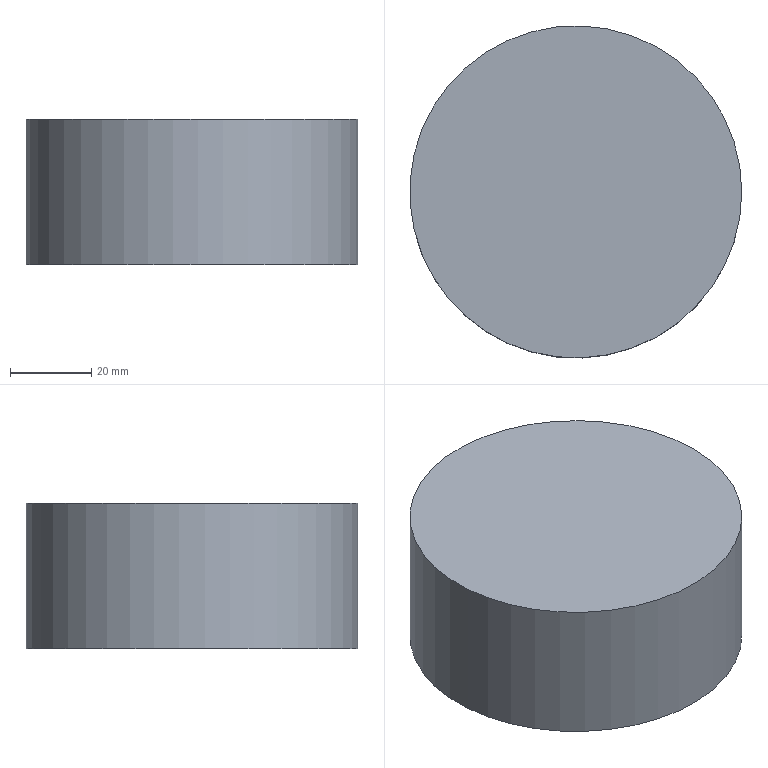Component | NX | SCREW_PLUG | 1 solid | 7 faces | box 81.95 x 81.95 x 36 mm | volume 189778 mm3 | cylinder 3 | plane 2 | cone 2 | commonest cylinder face diameters 4 x2 81.945 x1
STEP:
#1=CARTESIAN_POINT('',(0.,0.,0.));
#2=DIRECTION('',(0.,0.,1.));
#3=DIRECTION('',(1.,0.,0.));
#4=AXIS2_PLACEMENT_3D('',#1,#2,#3);
#5=CARTESIAN_POINT('',(122.222,-116.649,-169.615));
#6=VERTEX_POINT('',#5);
#7=CARTESIAN_POINT('',(81.249,-116.649,-169.615));
#8=DIRECTION('',(0.,0.,-1.));
#9=DIRECTION('',(1.,0.,0.));
#10=AXIS2_PLACEMENT_3D('',#7,#8,#9);
#11=CIRCLE('',#10,40.973);
#12=CARTESIAN_POINT('',(81.249,-116.649,-169.615));
#13=DIRECTION('',(0.,0.,1.));
#14=DIRECTION('',(1.,0.,0.));
#15=AXIS2_PLACEMENT_3D('',#12,#13,#14);
#16=PLANE('',#15);
#17=CARTESIAN_POINT('',(40.973,0.));
#18=CARTESIAN_POINT('',(40.973,-70.967));
#19=CARTESIAN_POINT('',(-20.486,-35.483));
#20=CARTESIAN_POINT('',(-81.945,-0.));
#21=CARTESIAN_POINT('',(-20.486,35.483));
#22=CARTESIAN_POINT('',(40.973,70.967));
#23=CARTESIAN_POINT('',(40.973,0.));
#24=(BOUNDED_CURVE()B_SPLINE_CURVE(2,(#17,#18,#19,#20,#21,#22,#23),.UNSPECIFIED.,.T.,.F.)B_SPLINE_CURVE_WITH_KNOTS((1,2,2,2,2,1),(-2.094,0.,2.094,4.189,6.283,8.378),.UNSPECIFIED.)CURVE()GEOMETRIC_REPRESENTATION_ITEM()RATIONAL_B_SPLINE_CURVE((1.,0.5,1.,0.5,1.,0.5,1.))REPRESENTATION_ITEM(''));
#25=(GEOMETRIC_REPRESENTATION_CONTEXT(2)PARAMETRIC_REPRESENTATION_CONTEXT()REPRESENTATION_CONTEXT('',''));
#26=DEFINITIONAL_REPRESENTATION('',(#24),#25);
#27=PCURVE('',#16,#26);
#28=CARTESIAN_POINT('',(81.249,-116.649,-205.615));
#29=DIRECTION('',(0.,0.,1.));
#30=DIRECTION('',(1.,0.,0.));
#31=AXIS2_PLACEMENT_3D('',#28,#29,#30);
#32=CYLINDRICAL_SURFACE('',#31,40.973);
#33=CARTESIAN_POINT('',(6.283,36.));
#34=DIRECTION('',(-1.,0.));
#35=VECTOR('',#34,1.);
#36=LINE('',#33,#35);
#37=(GEOMETRIC_REPRESENTATION_CONTEXT(2)PARAMETRIC_REPRESENTATION_CONTEXT()REPRESENTATION_CONTEXT('',''));
#38=DEFINITIONAL_REPRESENTATION('',(#36),#37);
#39=PCURVE('',#32,#38);
#40=SURFACE_CURVE('',#11,(#27,#39),.PCURVE_S1.);
#41=EDGE_CURVE('',#6,#6,#40,.T.);
#42=ORIENTED_EDGE('',*,*,#41,.F.);
#43=EDGE_LOOP('',(#42));
#44=FACE_BOUND('',#43,.T.);
#45=ADVANCED_FACE('',(#44),#16,.T.);
#46=CARTESIAN_POINT('',(62.999,-116.649,-205.615));
#47=VERTEX_POINT('',#46);
#48=CARTESIAN_POINT('',(60.999,-116.649,-205.615));
#49=DIRECTION('',(0.,0.,1.));
#50=DIRECTION('',(1.,0.,0.));
#51=AXIS2_PLACEMENT_3D('',#48,#49,#50);
#52=CIRCLE('',#51,2.);
#53=CARTESIAN_POINT('',(81.249,-116.649,-205.615));
#54=DIRECTION('',(0.,0.,-1.));
#55=DIRECTION('',(-1.,0.,0.));
#56=AXIS2_PLACEMENT_3D('',#53,#54,#55);
#57=PLANE('',#56);
#58=CARTESIAN_POINT('',(18.25,0.));
#59=CARTESIAN_POINT('',(18.25,3.464));
#60=CARTESIAN_POINT('',(21.25,1.732));
#61=CARTESIAN_POINT('',(24.25,0.));
#62=CARTESIAN_POINT('',(21.25,-1.732));
#63=CARTESIAN_POINT('',(18.25,-3.464));
#64=CARTESIAN_POINT('',(18.25,0.));
#65=(BOUNDED_CURVE()B_SPLINE_CURVE(2,(#58,#59,#60,#61,#62,#63,#64),.UNSPECIFIED.,.T.,.F.)B_SPLINE_CURVE_WITH_KNOTS((1,2,2,2,2,1),(-2.094,0.,2.094,4.189,6.283,8.378),.UNSPECIFIED.)CURVE()GEOMETRIC_REPRESENTATION_ITEM()RATIONAL_B_SPLINE_CURVE((1.,0.5,1.,0.5,1.,0.5,1.))REPRESENTATION_ITEM(''));
#66=(GEOMETRIC_REPRESENTATION_CONTEXT(2)PARAMETRIC_REPRESENTATION_CONTEXT()REPRESENTATION_CONTEXT('',''));
#67=DEFINITIONAL_REPRESENTATION('',(#65),#66);
#68=PCURVE('',#57,#67);
#69=CARTESIAN_POINT('',(60.999,-116.649,-205.615));
#70=DIRECTION('',(0.,0.,1.));
#71=DIRECTION('',(1.,0.,0.));
#72=AXIS2_PLACEMENT_3D('',#69,#70,#71);
#73=CYLINDRICAL_SURFACE('',#72,2.);
#74=CARTESIAN_POINT('',(0.,0.));
#75=DIRECTION('',(1.,0.));
#76=VECTOR('',#75,1.);
#77=LINE('',#74,#76);
#78=(GEOMETRIC_REPRESENTATION_CONTEXT(2)PARAMETRIC_REPRESENTATION_CONTEXT()REPRESENTATION_CONTEXT('',''));
#79=DEFINITIONAL_REPRESENTATION('',(#77),#78);
#80=PCURVE('',#73,#79);
#81=SURFACE_CURVE('',#52,(#68,#80),.PCURVE_S1.);
#82=EDGE_CURVE('',#47,#47,#81,.T.);
#83=ORIENTED_EDGE('',*,*,#82,.T.);
#84=EDGE_LOOP('',(#83));
#85=FACE_BOUND('',#84,.T.);
#86=CARTESIAN_POINT('',(103.499,-116.649,-205.615));
#87=VERTEX_POINT('',#86);
#88=CARTESIAN_POINT('',(101.499,-116.649,-205.615));
#89=DIRECTION('',(0.,0.,1.));
#90=DIRECTION('',(1.,0.,0.));
#91=AXIS2_PLACEMENT_3D('',#88,#89,#90);
#92=CIRCLE('',#91,2.);
#93=CARTESIAN_POINT('',(-22.25,0.));
#94=CARTESIAN_POINT('',(-22.25,3.464));
#95=CARTESIAN_POINT('',(-19.25,1.732));
#96=CARTESIAN_POINT('',(-16.25,0.));
#97=CARTESIAN_POINT('',(-19.25,-1.732));
#98=CARTESIAN_POINT('',(-22.25,-3.464));
#99=CARTESIAN_POINT('',(-22.25,0.));
#100=(BOUNDED_CURVE()B_SPLINE_CURVE(2,(#93,#94,#95,#96,#97,#98,#99),.UNSPECIFIED.,.T.,.F.)B_SPLINE_CURVE_WITH_KNOTS((1,2,2,2,2,1),(-2.094,0.,2.094,4.189,6.283,8.378),.UNSPECIFIED.)CURVE()GEOMETRIC_REPRESENTATION_ITEM()RATIONAL_B_SPLINE_CURVE((1.,0.5,1.,0.5,1.,0.5,1.))REPRESENTATION_ITEM(''));
#101=(GEOMETRIC_REPRESENTATION_CONTEXT(2)PARAMETRIC_REPRESENTATION_CONTEXT()REPRESENTATION_CONTEXT('',''));
#102=DEFINITIONAL_REPRESENTATION('',(#100),#101);
#103=PCURVE('',#57,#102);
#104=CARTESIAN_POINT('',(101.499,-116.649,-205.615));
#105=DIRECTION('',(0.,0.,1.));
#106=DIRECTION('',(1.,0.,0.));
#107=AXIS2_PLACEMENT_3D('',#104,#105,#106);
#108=CYLINDRICAL_SURFACE('',#107,2.);
#109=CARTESIAN_POINT('',(0.,0.));
#110=DIRECTION('',(1.,0.));
#111=VECTOR('',#110,1.);
#112=LINE('',#109,#111);
#113=(GEOMETRIC_REPRESENTATION_CONTEXT(2)PARAMETRIC_REPRESENTATION_CONTEXT()REPRESENTATION_CONTEXT('',''));
#114=DEFINITIONAL_REPRESENTATION('',(#112),#113);
#115=PCURVE('',#108,#114);
#116=SURFACE_CURVE('',#92,(#103,#115),.PCURVE_S1.);
#117=EDGE_CURVE('',#87,#87,#116,.T.);
#118=ORIENTED_EDGE('',*,*,#117,.T.);
#119=EDGE_LOOP('',(#118));
#120=FACE_BOUND('',#119,.T.);
#121=CARTESIAN_POINT('',(122.222,-116.649,-205.615));
#122=VERTEX_POINT('',#121);
#123=CARTESIAN_POINT('',(81.249,-116.649,-205.615));
#124=DIRECTION('',(0.,0.,1.));
#125=DIRECTION('',(1.,0.,0.));
#126=AXIS2_PLACEMENT_3D('',#123,#124,#125);
#127=CIRCLE('',#126,40.973);
#128=CARTESIAN_POINT('',(-40.973,0.));
#129=CARTESIAN_POINT('',(-40.973,70.967));
#130=CARTESIAN_POINT('',(20.486,35.483));
#131=CARTESIAN_POINT('',(81.945,0.));
#132=CARTESIAN_POINT('',(20.486,-35.483));
#133=CARTESIAN_POINT('',(-40.973,-70.967));
#134=CARTESIAN_POINT('',(-40.973,0.));
#135=(BOUNDED_CURVE()B_SPLINE_CURVE(2,(#128,#129,#130,#131,#132,#133,#134),.UNSPECIFIED.,.T.,.F.)B_SPLINE_CURVE_WITH_KNOTS((1,2,2,2,2,1),(-2.094,0.,2.094,4.189,6.283,8.378),.UNSPECIFIED.)CURVE()GEOMETRIC_REPRESENTATION_ITEM()RATIONAL_B_SPLINE_CURVE((1.,0.5,1.,0.5,1.,0.5,1.))REPRESENTATION_ITEM(''));
#136=(GEOMETRIC_REPRESENTATION_CONTEXT(2)PARAMETRIC_REPRESENTATION_CONTEXT()REPRESENTATION_CONTEXT('',''));
#137=DEFINITIONAL_REPRESENTATION('',(#135),#136);
#138=PCURVE('',#57,#137);
#139=CARTESIAN_POINT('',(0.,0.));
#140=DIRECTION('',(1.,0.));
#141=VECTOR('',#140,1.);
#142=LINE('',#139,#141);
#143=(GEOMETRIC_REPRESENTATION_CONTEXT(2)PARAMETRIC_REPRESENTATION_CONTEXT()REPRESENTATION_CONTEXT('',''));
#144=DEFINITIONAL_REPRESENTATION('',(#142),#143);
#145=PCURVE('',#32,#144);
#146=SURFACE_CURVE('',#127,(#138,#145),.PCURVE_S1.);
#147=EDGE_CURVE('',#122,#122,#146,.T.);
#148=ORIENTED_EDGE('',*,*,#147,.F.);
#149=EDGE_LOOP('',(#148));
#150=FACE_BOUND('',#149,.T.);
#151=ADVANCED_FACE('',(#85,#120,#150),#57,.T.);
#152=ORIENTED_EDGE('',*,*,#41,.T.);
#153=CARTESIAN_POINT('',(122.222,-116.649,-205.615));
#154=CARTESIAN_POINT('',(122.222,-116.649,-169.615));
#155=B_SPLINE_CURVE_WITH_KNOTS('',1,(#153,#154),.UNSPECIFIED.,.F.,.F.,(2,2),(0.,36.),.PIECEWISE_BEZIER_KNOTS.);
#156=CARTESIAN_POINT('',(0.,0.));
#157=DIRECTION('',(0.,1.));
#158=VECTOR('',#157,1.);
#159=LINE('',#156,#158);
#160=(GEOMETRIC_REPRESENTATION_CONTEXT(2)PARAMETRIC_REPRESENTATION_CONTEXT()REPRESENTATION_CONTEXT('',''));
#161=DEFINITIONAL_REPRESENTATION('',(#159),#160);
#162=PCURVE('',#32,#161);
#163=CARTESIAN_POINT('',(6.283,0.));
#164=DIRECTION('',(0.,1.));
#165=VECTOR('',#164,1.);
#166=LINE('',#163,#165);
#167=(GEOMETRIC_REPRESENTATION_CONTEXT(2)PARAMETRIC_REPRESENTATION_CONTEXT()REPRESENTATION_CONTEXT('',''));
#168=DEFINITIONAL_REPRESENTATION('',(#166),#167);
#169=PCURVE('',#32,#168);
#170=SEAM_CURVE('',#155,(#162,#169),.PCURVE_S1.);
#171=EDGE_CURVE('',#122,#6,#170,.T.);
#172=ORIENTED_EDGE('',*,*,#171,.F.);
#173=ORIENTED_EDGE('',*,*,#147,.T.);
#174=ORIENTED_EDGE('',*,*,#171,.T.);
#175=EDGE_LOOP('',(#152,#172,#173,#174));
#176=FACE_BOUND('',#175,.T.);
#177=ADVANCED_FACE('',(#176),#32,.T.);
#178=CARTESIAN_POINT('',(99.499,-116.649,-202.615));
#179=VERTEX_POINT('',#178);
#180=CARTESIAN_POINT('',(103.499,-116.649,-202.615));
#181=VERTEX_POINT('',#180);
#182=CARTESIAN_POINT('',(101.499,-116.649,-202.615));
#183=DIRECTION('',(0.,0.,-1.));
#184=DIRECTION('',(1.,0.,0.));
#185=AXIS2_PLACEMENT_3D('',#182,#183,#184);
#186=CIRCLE('',#185,2.);
#187=CARTESIAN_POINT('',(101.499,-116.649,-202.615));
#188=DIRECTION('',(0.,0.,-1.));
#189=DIRECTION('',(-1.,0.,0.));
#190=AXIS2_PLACEMENT_3D('',#187,#188,#189);
#191=CONICAL_SURFACE('',#190,2.,1.03);
#192=CARTESIAN_POINT('',(-3.142,0.));
#193=DIRECTION('',(1.,0.));
#194=VECTOR('',#193,1.);
#195=LINE('',#192,#194);
#196=(GEOMETRIC_REPRESENTATION_CONTEXT(2)PARAMETRIC_REPRESENTATION_CONTEXT()REPRESENTATION_CONTEXT('',''));
#197=DEFINITIONAL_REPRESENTATION('',(#195),#196);
#198=PCURVE('',#191,#197);
#199=CARTESIAN_POINT('',(6.283,3.));
#200=DIRECTION('',(-1.,0.));
#201=VECTOR('',#200,1.);
#202=LINE('',#199,#201);
#203=(GEOMETRIC_REPRESENTATION_CONTEXT(2)PARAMETRIC_REPRESENTATION_CONTEXT()REPRESENTATION_CONTEXT('',''));
#204=DEFINITIONAL_REPRESENTATION('',(#202),#203);
#205=PCURVE('',#108,#204);
#206=SURFACE_CURVE('',#186,(#198,#205),.PCURVE_S1.);
#207=EDGE_CURVE('',#179,#181,#206,.T.);
#208=ORIENTED_EDGE('',*,*,#207,.F.);
#209=CARTESIAN_POINT('',(101.499,-116.649,-201.413));
#210=VERTEX_POINT('',#209);
#211=CARTESIAN_POINT('',(101.499,-116.649,-201.413));
#212=CARTESIAN_POINT('',(99.499,-116.649,-202.615));
#213=B_SPLINE_CURVE_WITH_KNOTS('',1,(#211,#212),.UNSPECIFIED.,.F.,.F.,(2,2),(-2.333,0.),.PIECEWISE_BEZIER_KNOTS.);
#214=CARTESIAN_POINT('',(0.,0.));
#215=DIRECTION('',(0.,1.));
#216=VECTOR('',#215,1.);
#217=LINE('',#214,#216);
#218=(GEOMETRIC_REPRESENTATION_CONTEXT(2)PARAMETRIC_REPRESENTATION_CONTEXT()REPRESENTATION_CONTEXT('',''));
#219=DEFINITIONAL_REPRESENTATION('',(#217),#218);
#220=PCURVE('',#191,#219);
#221=CARTESIAN_POINT('',(6.283,0.));
#222=DIRECTION('',(0.,1.));
#223=VECTOR('',#222,1.);
#224=LINE('',#221,#223);
#225=(GEOMETRIC_REPRESENTATION_CONTEXT(2)PARAMETRIC_REPRESENTATION_CONTEXT()REPRESENTATION_CONTEXT('',''));
#226=DEFINITIONAL_REPRESENTATION('',(#224),#225);
#227=PCURVE('',#191,#226);
#228=SEAM_CURVE('',#213,(#220,#227),.PCURVE_S1.);
#229=EDGE_CURVE('',#210,#179,#228,.T.);
#230=ORIENTED_EDGE('',*,*,#229,.F.);
#231=ORIENTED_EDGE('',*,*,#229,.T.);
#232=CARTESIAN_POINT('',(101.499,-116.649,-202.615));
#233=DIRECTION('',(0.,0.,-1.));
#234=DIRECTION('',(1.,0.,0.));
#235=AXIS2_PLACEMENT_3D('',#232,#233,#234);
#236=CIRCLE('',#235,2.);
#237=CARTESIAN_POINT('',(3.142,0.));
#238=DIRECTION('',(1.,0.));
#239=VECTOR('',#238,1.);
#240=LINE('',#237,#239);
#241=(GEOMETRIC_REPRESENTATION_CONTEXT(2)PARAMETRIC_REPRESENTATION_CONTEXT()REPRESENTATION_CONTEXT('',''));
#242=DEFINITIONAL_REPRESENTATION('',(#240),#241);
#243=PCURVE('',#191,#242);
#244=CARTESIAN_POINT('',(6.283,3.));
#245=DIRECTION('',(-1.,0.));
#246=VECTOR('',#245,1.);
#247=LINE('',#244,#246);
#248=(GEOMETRIC_REPRESENTATION_CONTEXT(2)PARAMETRIC_REPRESENTATION_CONTEXT()REPRESENTATION_CONTEXT('',''));
#249=DEFINITIONAL_REPRESENTATION('',(#247),#248);
#250=PCURVE('',#108,#249);
#251=SURFACE_CURVE('',#236,(#243,#250),.PCURVE_S1.);
#252=EDGE_CURVE('',#181,#179,#251,.T.);
#253=ORIENTED_EDGE('',*,*,#252,.F.);
#254=EDGE_LOOP('',(#208,#230,#231,#253));
#255=FACE_BOUND('',#254,.F.);
#256=ADVANCED_FACE('',(#255),#191,.F.);
#257=ORIENTED_EDGE('',*,*,#207,.T.);
#258=CARTESIAN_POINT('',(103.499,-116.649,-205.615));
#259=CARTESIAN_POINT('',(103.499,-116.649,-202.615));
#260=B_SPLINE_CURVE_WITH_KNOTS('',1,(#258,#259),.UNSPECIFIED.,.F.,.F.,(2,2),(0.,3.),.PIECEWISE_BEZIER_KNOTS.);
#261=CARTESIAN_POINT('',(0.,0.));
#262=DIRECTION('',(0.,1.));
#263=VECTOR('',#262,1.);
#264=LINE('',#261,#263);
#265=(GEOMETRIC_REPRESENTATION_CONTEXT(2)PARAMETRIC_REPRESENTATION_CONTEXT()REPRESENTATION_CONTEXT('',''));
#266=DEFINITIONAL_REPRESENTATION('',(#264),#265);
#267=PCURVE('',#108,#266);
#268=CARTESIAN_POINT('',(6.283,0.));
#269=DIRECTION('',(0.,1.));
#270=VECTOR('',#269,1.);
#271=LINE('',#268,#270);
#272=(GEOMETRIC_REPRESENTATION_CONTEXT(2)PARAMETRIC_REPRESENTATION_CONTEXT()REPRESENTATION_CONTEXT('',''));
#273=DEFINITIONAL_REPRESENTATION('',(#271),#272);
#274=PCURVE('',#108,#273);
#275=SEAM_CURVE('',#260,(#267,#274),.PCURVE_S1.);
#276=EDGE_CURVE('',#87,#181,#275,.T.);
#277=ORIENTED_EDGE('',*,*,#276,.F.);
#278=ORIENTED_EDGE('',*,*,#117,.T.);
#279=ORIENTED_EDGE('',*,*,#276,.T.);
#280=ORIENTED_EDGE('',*,*,#252,.T.);
#281=EDGE_LOOP('',(#257,#277,#278,#279,#280));
#282=FACE_BOUND('',#281,.F.);
#283=ADVANCED_FACE('',(#282),#108,.F.);
#284=CARTESIAN_POINT('',(58.999,-116.649,-202.615));
#285=VERTEX_POINT('',#284);
#286=CARTESIAN_POINT('',(62.999,-116.649,-202.615));
#287=VERTEX_POINT('',#286);
#288=CARTESIAN_POINT('',(60.999,-116.649,-202.615));
#289=DIRECTION('',(0.,0.,-1.));
#290=DIRECTION('',(1.,0.,0.));
#291=AXIS2_PLACEMENT_3D('',#288,#289,#290);
#292=CIRCLE('',#291,2.);
#293=CARTESIAN_POINT('',(60.999,-116.649,-202.615));
#294=DIRECTION('',(0.,0.,-1.));
#295=DIRECTION('',(-1.,0.,0.));
#296=AXIS2_PLACEMENT_3D('',#293,#294,#295);
#297=CONICAL_SURFACE('',#296,2.,1.03);
#298=CARTESIAN_POINT('',(-3.142,0.));
#299=DIRECTION('',(1.,0.));
#300=VECTOR('',#299,1.);
#301=LINE('',#298,#300);
#302=(GEOMETRIC_REPRESENTATION_CONTEXT(2)PARAMETRIC_REPRESENTATION_CONTEXT()REPRESENTATION_CONTEXT('',''));
#303=DEFINITIONAL_REPRESENTATION('',(#301),#302);
#304=PCURVE('',#297,#303);
#305=CARTESIAN_POINT('',(6.283,3.));
#306=DIRECTION('',(-1.,0.));
#307=VECTOR('',#306,1.);
#308=LINE('',#305,#307);
#309=(GEOMETRIC_REPRESENTATION_CONTEXT(2)PARAMETRIC_REPRESENTATION_CONTEXT()REPRESENTATION_CONTEXT('',''));
#310=DEFINITIONAL_REPRESENTATION('',(#308),#309);
#311=PCURVE('',#73,#310);
#312=SURFACE_CURVE('',#292,(#304,#311),.PCURVE_S1.);
#313=EDGE_CURVE('',#285,#287,#312,.T.);
#314=ORIENTED_EDGE('',*,*,#313,.F.);
#315=CARTESIAN_POINT('',(60.999,-116.649,-201.413));
#316=VERTEX_POINT('',#315);
#317=CARTESIAN_POINT('',(60.999,-116.649,-201.413));
#318=CARTESIAN_POINT('',(58.999,-116.649,-202.615));
#319=B_SPLINE_CURVE_WITH_KNOTS('',1,(#317,#318),.UNSPECIFIED.,.F.,.F.,(2,2),(-2.333,0.),.PIECEWISE_BEZIER_KNOTS.);
#320=CARTESIAN_POINT('',(0.,0.));
#321=DIRECTION('',(0.,1.));
#322=VECTOR('',#321,1.);
#323=LINE('',#320,#322);
#324=(GEOMETRIC_REPRESENTATION_CONTEXT(2)PARAMETRIC_REPRESENTATION_CONTEXT()REPRESENTATION_CONTEXT('',''));
#325=DEFINITIONAL_REPRESENTATION('',(#323),#324);
#326=PCURVE('',#297,#325);
#327=CARTESIAN_POINT('',(6.283,0.));
#328=DIRECTION('',(0.,1.));
#329=VECTOR('',#328,1.);
#330=LINE('',#327,#329);
#331=(GEOMETRIC_REPRESENTATION_CONTEXT(2)PARAMETRIC_REPRESENTATION_CONTEXT()REPRESENTATION_CONTEXT('',''));
#332=DEFINITIONAL_REPRESENTATION('',(#330),#331);
#333=PCURVE('',#297,#332);
#334=SEAM_CURVE('',#319,(#326,#333),.PCURVE_S1.);
#335=EDGE_CURVE('',#316,#285,#334,.T.);
#336=ORIENTED_EDGE('',*,*,#335,.F.);
#337=ORIENTED_EDGE('',*,*,#335,.T.);
#338=CARTESIAN_POINT('',(60.999,-116.649,-202.615));
#339=DIRECTION('',(0.,0.,-1.));
#340=DIRECTION('',(1.,0.,0.));
#341=AXIS2_PLACEMENT_3D('',#338,#339,#340);
#342=CIRCLE('',#341,2.);
#343=CARTESIAN_POINT('',(3.142,0.));
#344=DIRECTION('',(1.,0.));
#345=VECTOR('',#344,1.);
#346=LINE('',#343,#345);
#347=(GEOMETRIC_REPRESENTATION_CONTEXT(2)PARAMETRIC_REPRESENTATION_CONTEXT()REPRESENTATION_CONTEXT('',''));
#348=DEFINITIONAL_REPRESENTATION('',(#346),#347);
#349=PCURVE('',#297,#348);
#350=CARTESIAN_POINT('',(6.283,3.));
#351=DIRECTION('',(-1.,0.));
#352=VECTOR('',#351,1.);
#353=LINE('',#350,#352);
#354=(GEOMETRIC_REPRESENTATION_CONTEXT(2)PARAMETRIC_REPRESENTATION_CONTEXT()REPRESENTATION_CONTEXT('',''));
#355=DEFINITIONAL_REPRESENTATION('',(#353),#354);
#356=PCURVE('',#73,#355);
#357=SURFACE_CURVE('',#342,(#349,#356),.PCURVE_S1.);
#358=EDGE_CURVE('',#287,#285,#357,.T.);
#359=ORIENTED_EDGE('',*,*,#358,.F.);
#360=EDGE_LOOP('',(#314,#336,#337,#359));
#361=FACE_BOUND('',#360,.F.);
#362=ADVANCED_FACE('',(#361),#297,.F.);
#363=ORIENTED_EDGE('',*,*,#313,.T.);
#364=CARTESIAN_POINT('',(62.999,-116.649,-205.615));
#365=CARTESIAN_POINT('',(62.999,-116.649,-202.615));
#366=B_SPLINE_CURVE_WITH_KNOTS('',1,(#364,#365),.UNSPECIFIED.,.F.,.F.,(2,2),(0.,3.),.PIECEWISE_BEZIER_KNOTS.);
#367=CARTESIAN_POINT('',(0.,0.));
#368=DIRECTION('',(0.,1.));
#369=VECTOR('',#368,1.);
#370=LINE('',#367,#369);
#371=(GEOMETRIC_REPRESENTATION_CONTEXT(2)PARAMETRIC_REPRESENTATION_CONTEXT()REPRESENTATION_CONTEXT('',''));
#372=DEFINITIONAL_REPRESENTATION('',(#370),#371);
#373=PCURVE('',#73,#372);
#374=CARTESIAN_POINT('',(6.283,0.));
#375=DIRECTION('',(0.,1.));
#376=VECTOR('',#375,1.);
#377=LINE('',#374,#376);
#378=(GEOMETRIC_REPRESENTATION_CONTEXT(2)PARAMETRIC_REPRESENTATION_CONTEXT()REPRESENTATION_CONTEXT('',''));
#379=DEFINITIONAL_REPRESENTATION('',(#377),#378);
#380=PCURVE('',#73,#379);
#381=SEAM_CURVE('',#366,(#373,#380),.PCURVE_S1.);
#382=EDGE_CURVE('',#47,#287,#381,.T.);
#383=ORIENTED_EDGE('',*,*,#382,.F.);
#384=ORIENTED_EDGE('',*,*,#82,.T.);
#385=ORIENTED_EDGE('',*,*,#382,.T.);
#386=ORIENTED_EDGE('',*,*,#358,.T.);
#387=EDGE_LOOP('',(#363,#383,#384,#385,#386));
#388=FACE_BOUND('',#387,.F.);
#389=ADVANCED_FACE('',(#388),#73,.F.);
#390=CLOSED_SHELL('',(#45,#151,#177,#256,#283,#362,#389));
#391=MANIFOLD_SOLID_BREP('',#390);
#392=(LENGTH_UNIT()NAMED_UNIT(*)SI_UNIT(.MILLI.,.METRE.));
#393=UNCERTAINTY_MEASURE_WITH_UNIT(LENGTH_MEASURE(0.00001),#392,'','');
#394=(NAMED_UNIT(*)PLANE_ANGLE_UNIT()SI_UNIT($,.RADIAN.));
#395=(NAMED_UNIT(*)SI_UNIT($,.STERADIAN.)SOLID_ANGLE_UNIT());
#396=(GEOMETRIC_REPRESENTATION_CONTEXT(3)GLOBAL_UNCERTAINTY_ASSIGNED_CONTEXT((#393))GLOBAL_UNIT_ASSIGNED_CONTEXT((#392,#394,#395))REPRESENTATION_CONTEXT('',''));
#397=ADVANCED_BREP_SHAPE_REPRESENTATION('',(#4,#391),#396);